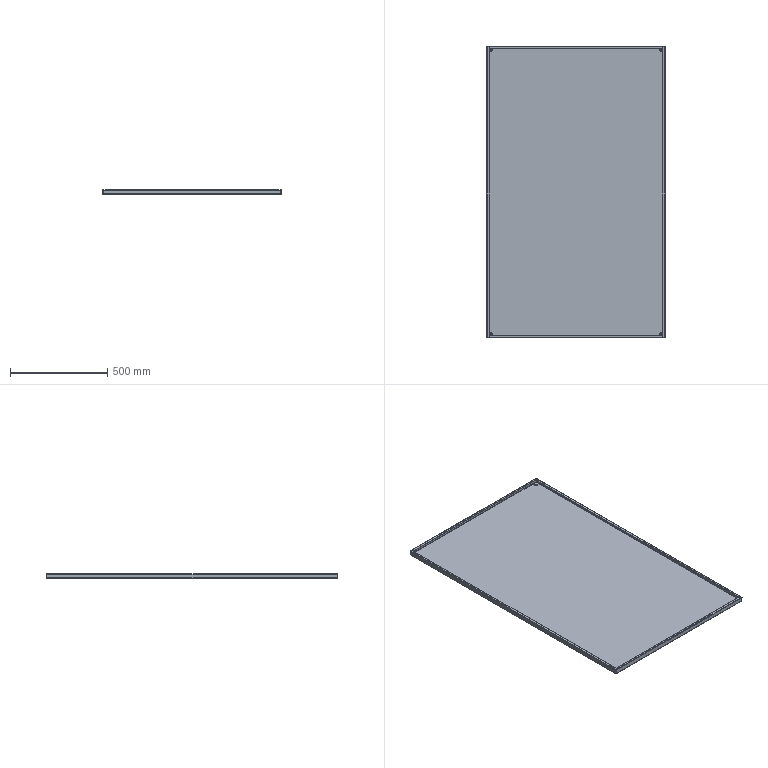Component | SolidWorks | AirFurnaceElectricalCabinet-RearSealingPlateAssembly-1_AirFurnaceElectricalCabinet-RearSealingPlate-1 | 1 solid | 94 faces | volume 2294459 mm3 | plane 54 | torus 16 | cylinder 16 | spline 8 | commonest cylinder face diameters 1.5 x8 4.5 x8